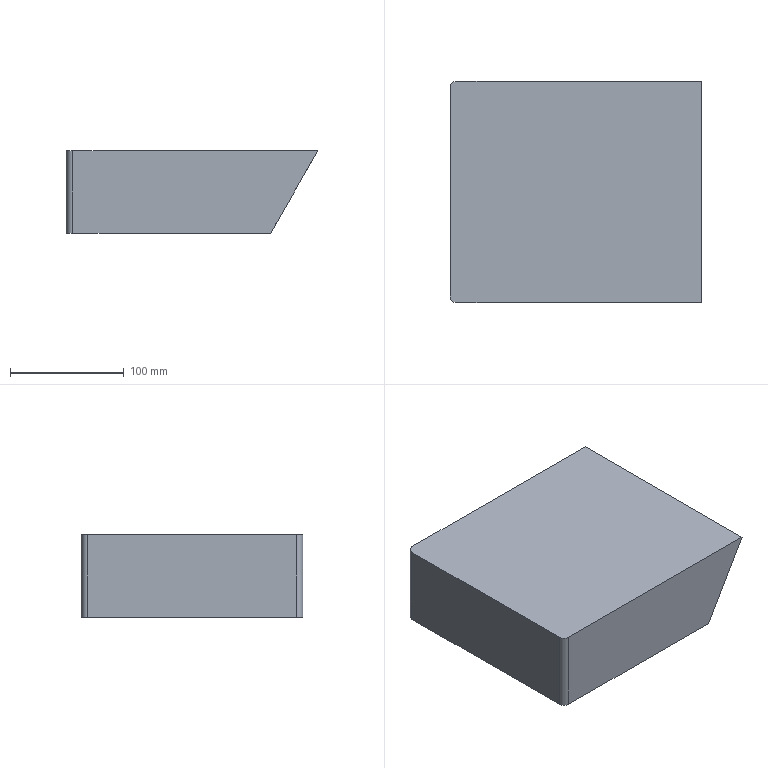Component | NX | SLIDE_COVER_LARGE | 1 solid | 20 faces | volume 484416 mm3 | plane 14 | cylinder 6 | commonest cylinder face diameters 3 x4 12 x2